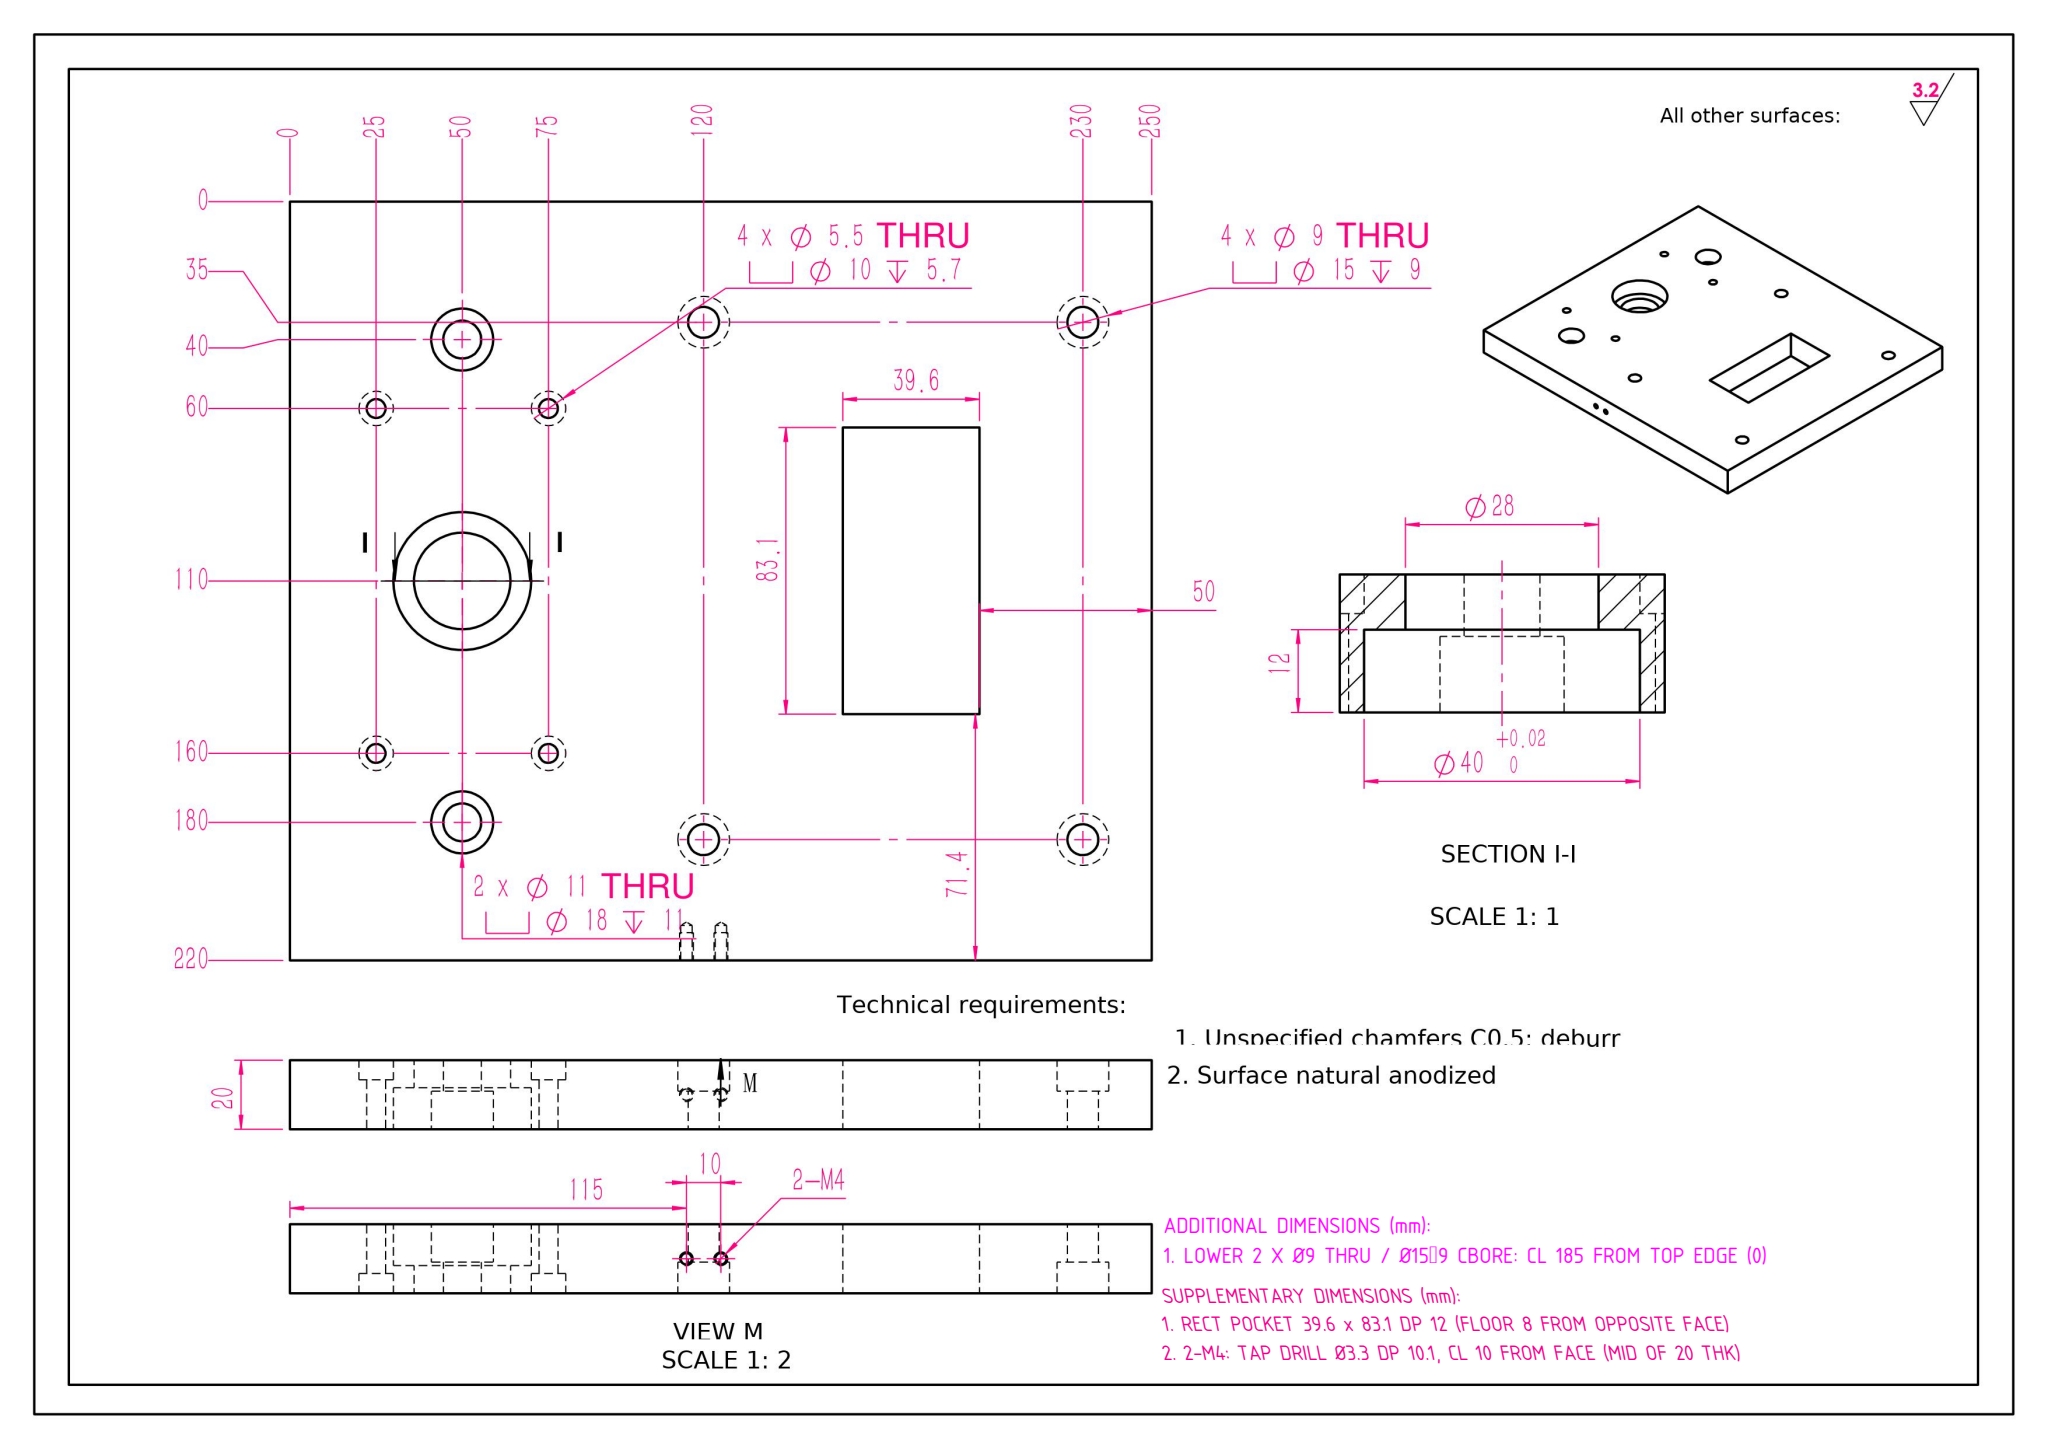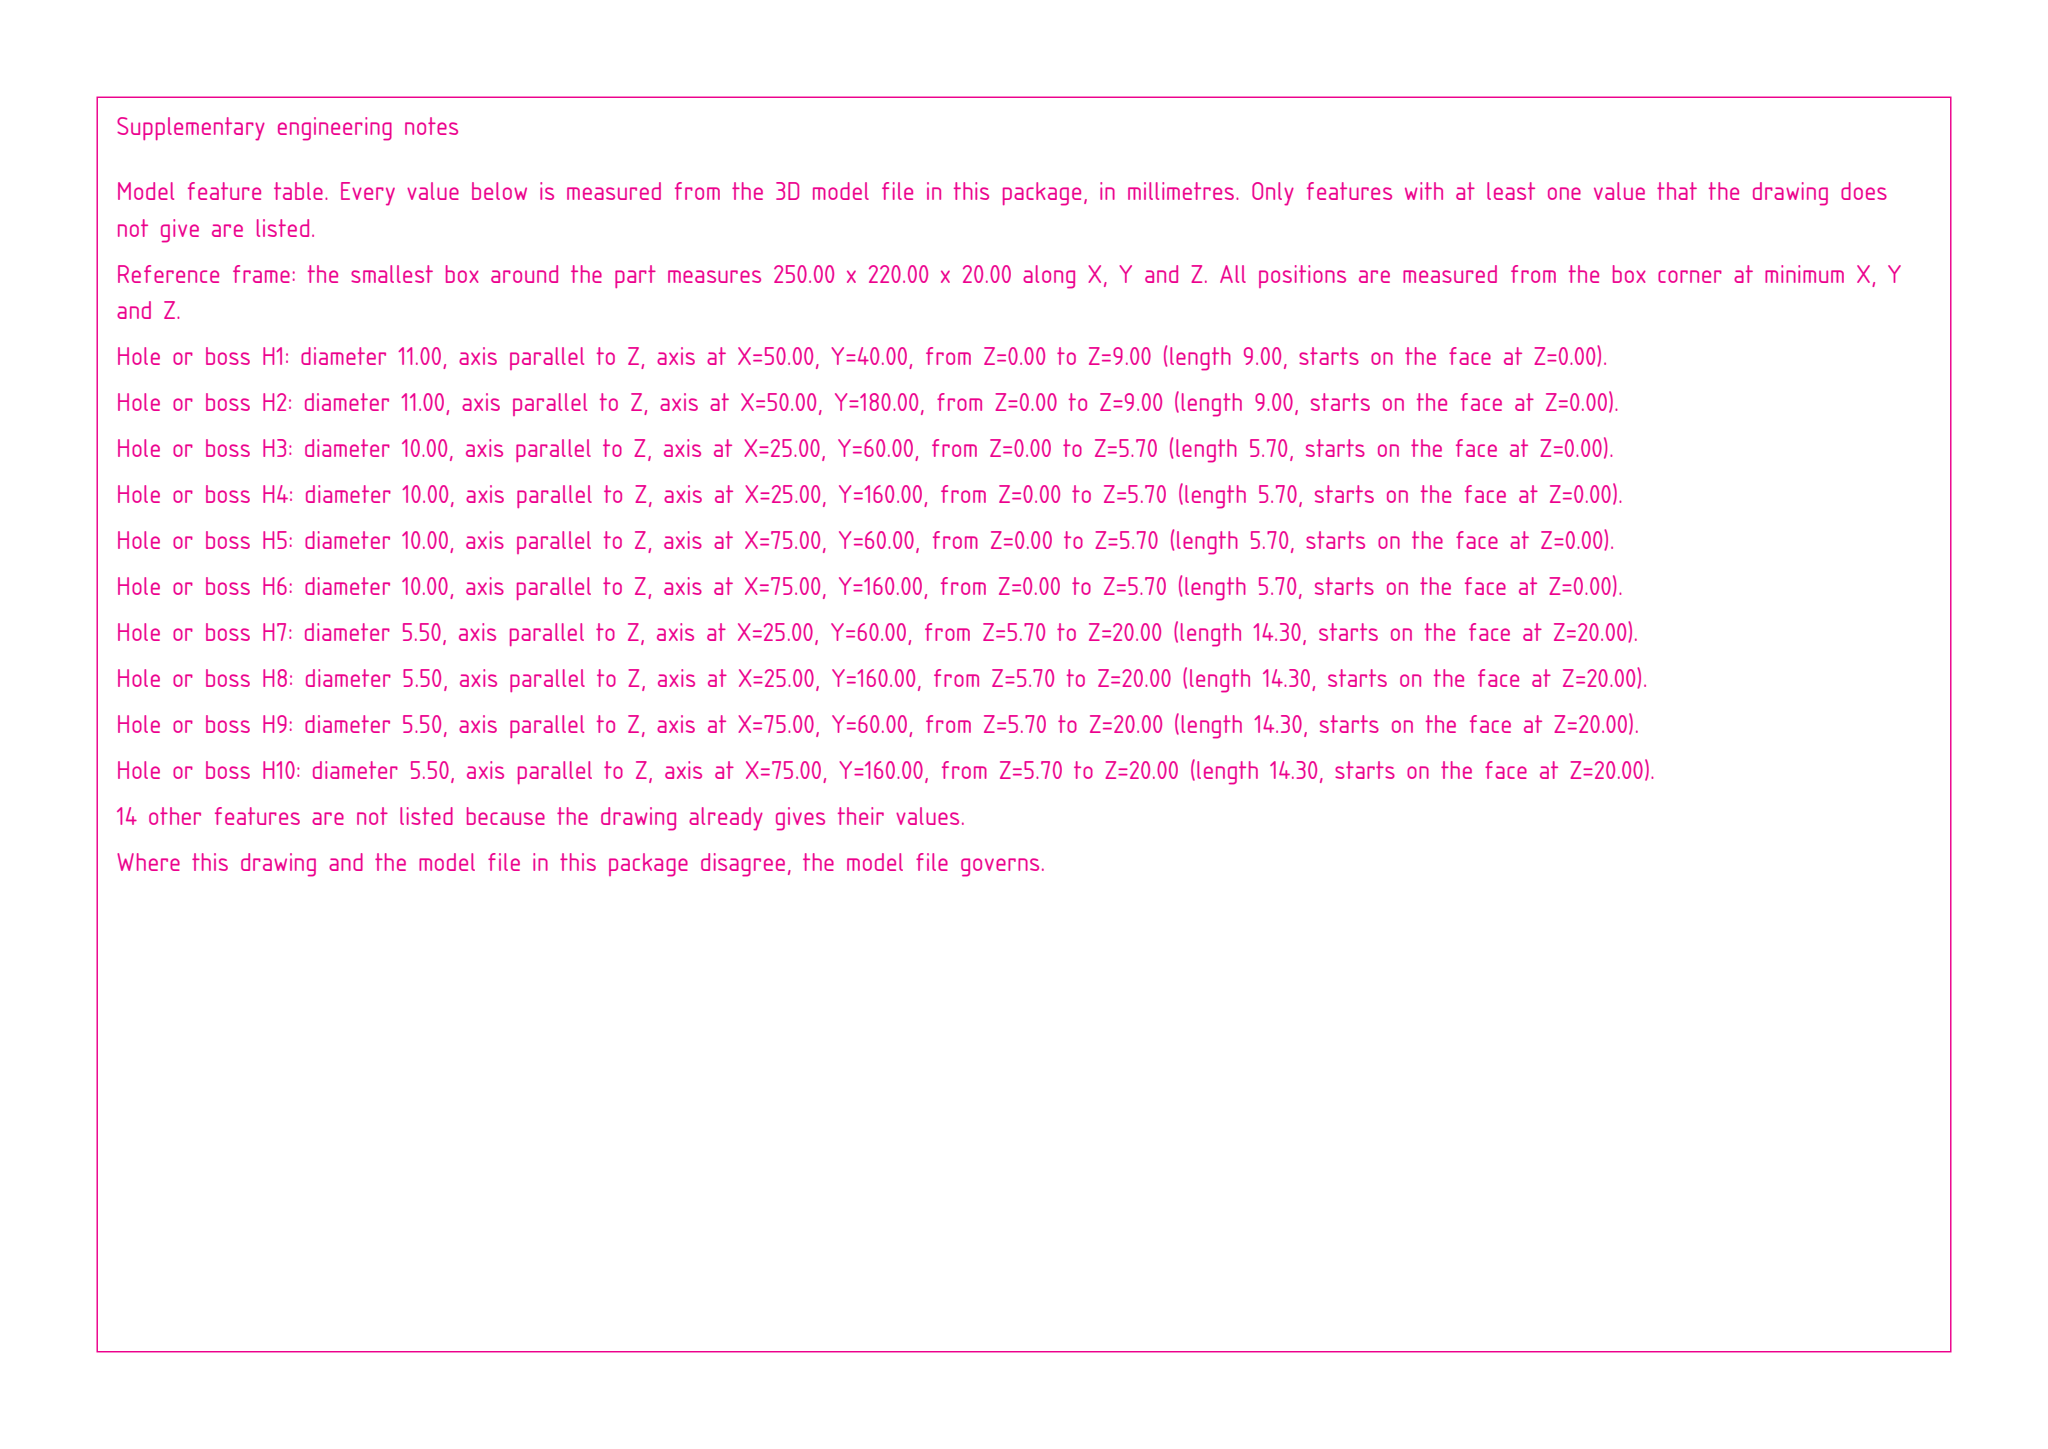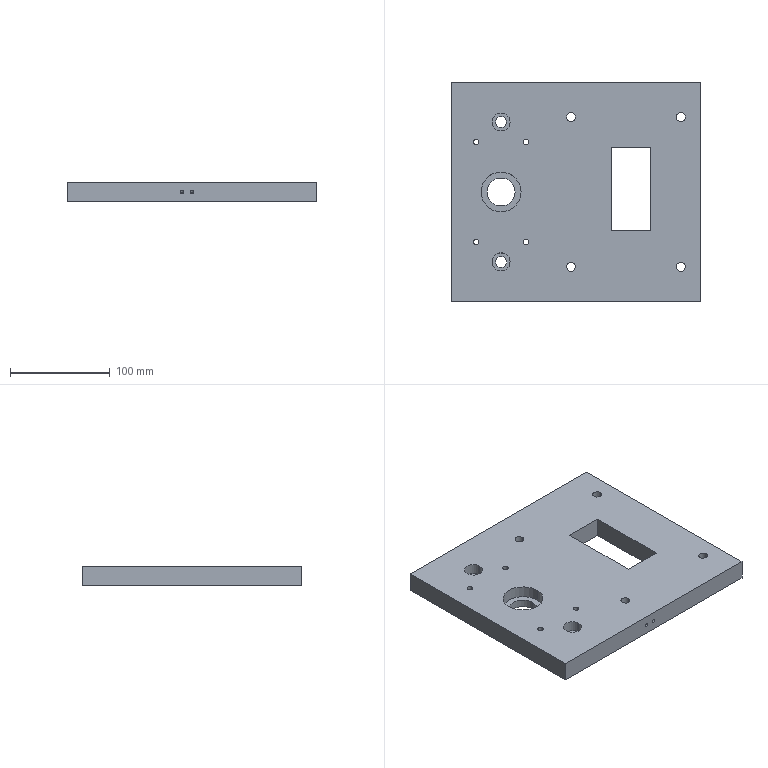Part | SolidWorks | mm | 1 solid | 73 faces | box 250 x 220 x 20 mm | volume 994277 mm3 | cylinder 48 | plane 21 | cone 4 | commonest cylinder face diameters 10 x8 5.5 x8 15 x8 9 x8 3.3 x4 18 x4 11 x4 28 x2
build123d program:
from build123d import *

# Parameters (mm, degrees)
SKETCH1_W                                            = 250
SKETCH1_H                                            = 220
BOSS_EXTRUDE1_DEPTH                                  = 20
HOLE_SIZE_ACCORDING_TO_HEXAGON_SOCKET_HE_D           = 11
HOLE_SIZE_ACCORDING_TO_HEXAGON_SOCKET_HE_CBORE_D     = 18
HOLE_SIZE_ACCORDING_TO_HEXAGON_SOCKET_HE_CBORE_DEPTH = 11
SKETCH7_R                                            = 20
CUT_EXTRUDE1_DEPTH                                   = 12
SKETCH8_R                                            = 14
CUT_EXTRUDE2_DEPTH                                   = 167.94
HOLE_SIZE_ACCORDING_TO_HEXAGON_SOCKE_2_D             = 9
HOLE_SIZE_ACCORDING_TO_HEXAGON_SOCKE_2_CBORE_D       = 15
HOLE_SIZE_ACCORDING_TO_HEXAGON_SOCKE_2_CBORE_DEPTH   = 9
HOLE_SIZE_ACCORDING_TO_HEXAGON_SOCKE_3_D             = 5.5
HOLE_SIZE_ACCORDING_TO_HEXAGON_SOCKE_3_CBORE_D       = 10
HOLE_SIZE_ACCORDING_TO_HEXAGON_SOCKE_3_CBORE_DEPTH   = 5.7
M4_TAPPED_HOLE1_D                                    = 3.3
M4_TAPPED_HOLE1_DEPTH                                = 10.1
M4_TAPPED_HOLE1_TIP                                  = 0.9914
SKETCH15_W                                           = 39.649
SKETCH15_H                                           = 83.129
CUT_EXTRUDE3_DEPTH                                   = 48


with BuildPart() as part:
    # Sketch1 → Boss-Extrude1 (new body)
    with BuildSketch(Plane.XY):
        Rectangle(SKETCH1_W, SKETCH1_H)
    extrude(amount=BOSS_EXTRUDE1_DEPTH)

    # Hole Size according to Hexagon Socket He (through all)
    with Locations(Plane.XY.offset(20)):
        with Locations((-75, 70), (-75, -70)):
            CounterBoreHole(HOLE_SIZE_ACCORDING_TO_HEXAGON_SOCKET_HE_D / 2, HOLE_SIZE_ACCORDING_TO_HEXAGON_SOCKET_HE_CBORE_D / 2, HOLE_SIZE_ACCORDING_TO_HEXAGON_SOCKET_HE_CBORE_DEPTH)

    # Sketch7 → Cut-Extrude1 (cut)
    with BuildSketch(Plane.XY.offset(20)):
        with Locations((-75, 0)):
            Circle(SKETCH7_R)
    extrude(amount=-CUT_EXTRUDE1_DEPTH, mode=Mode.SUBTRACT)

    # Sketch8 → Cut-Extrude2 (cut, through all)
    with BuildSketch(Plane.XY.offset(8)):
        with Locations((-75, 0)):
            Circle(SKETCH8_R)
    extrude(amount=-CUT_EXTRUDE2_DEPTH, mode=Mode.SUBTRACT)

    # Hole Size according to Hexagon Socke 2 (through all)
    with Locations(Plane(origin=(0, 0, 0), x_dir=(-1, 0, 0), z_dir=(0, 0, -1))):
        with Locations((-105, 75), (-105, -75), (5, 75), (5, -75)):
            CounterBoreHole(HOLE_SIZE_ACCORDING_TO_HEXAGON_SOCKE_2_D / 2, HOLE_SIZE_ACCORDING_TO_HEXAGON_SOCKE_2_CBORE_D / 2, HOLE_SIZE_ACCORDING_TO_HEXAGON_SOCKE_2_CBORE_DEPTH)

    # Hole Size according to Hexagon Socke 3 (through all)
    with Locations(Plane(origin=(0, 0, 0), x_dir=(-1, 0, 0), z_dir=(0, 0, -1))):
        with Locations((50, 50), (100, 50), (100, -50), (50, -50)):
            CounterBoreHole(HOLE_SIZE_ACCORDING_TO_HEXAGON_SOCKE_3_D / 2, HOLE_SIZE_ACCORDING_TO_HEXAGON_SOCKE_3_CBORE_D / 2, HOLE_SIZE_ACCORDING_TO_HEXAGON_SOCKE_3_CBORE_DEPTH)

    # M4 Tapped Hole1
    with Locations(Plane(origin=(0, -110, 0), x_dir=(-1, 0, 0), z_dir=(0, -1, 0))):
        with Locations((10, -10), (0, -10)):
            Hole(M4_TAPPED_HOLE1_D / 2, depth=M4_TAPPED_HOLE1_DEPTH)
            with Locations((0, 0, -(M4_TAPPED_HOLE1_DEPTH + M4_TAPPED_HOLE1_TIP / 2))):  # 118° drill point
                Cone(0, M4_TAPPED_HOLE1_D / 2, M4_TAPPED_HOLE1_TIP, mode=Mode.SUBTRACT)

    # Sketch15 → Cut-Extrude3 (cut)
    with BuildSketch(Plane.XY.offset(20)):
        with Locations((55.194, 2.929)):
            Rectangle(SKETCH15_W, SKETCH15_H)
    extrude(amount=-CUT_EXTRUDE3_DEPTH, mode=Mode.SUBTRACT)


solid = part.part